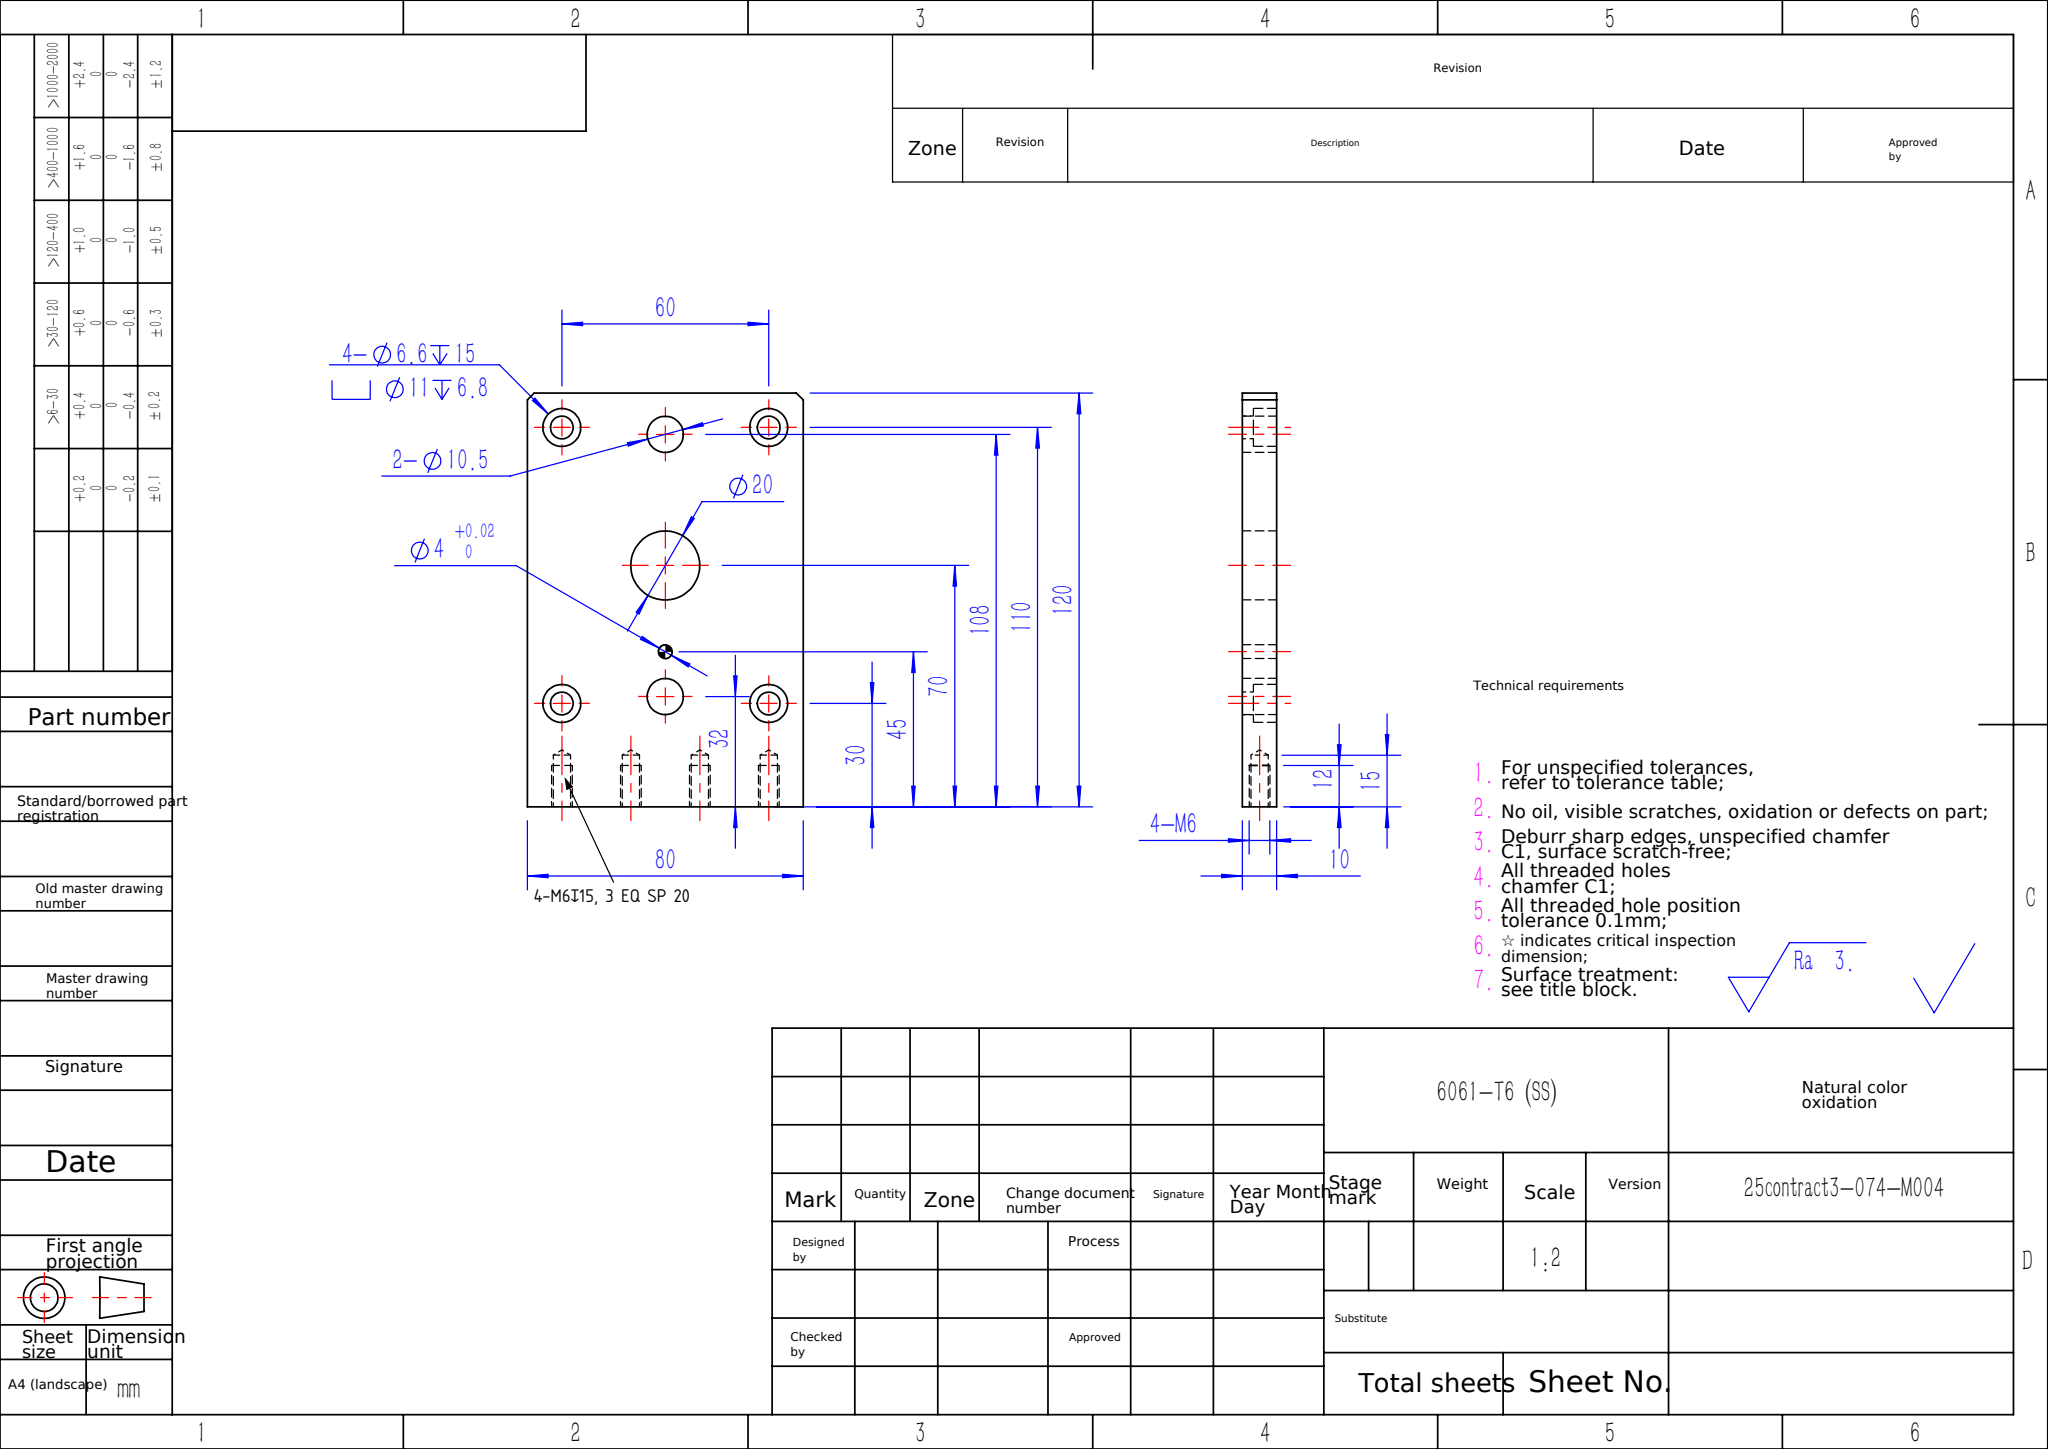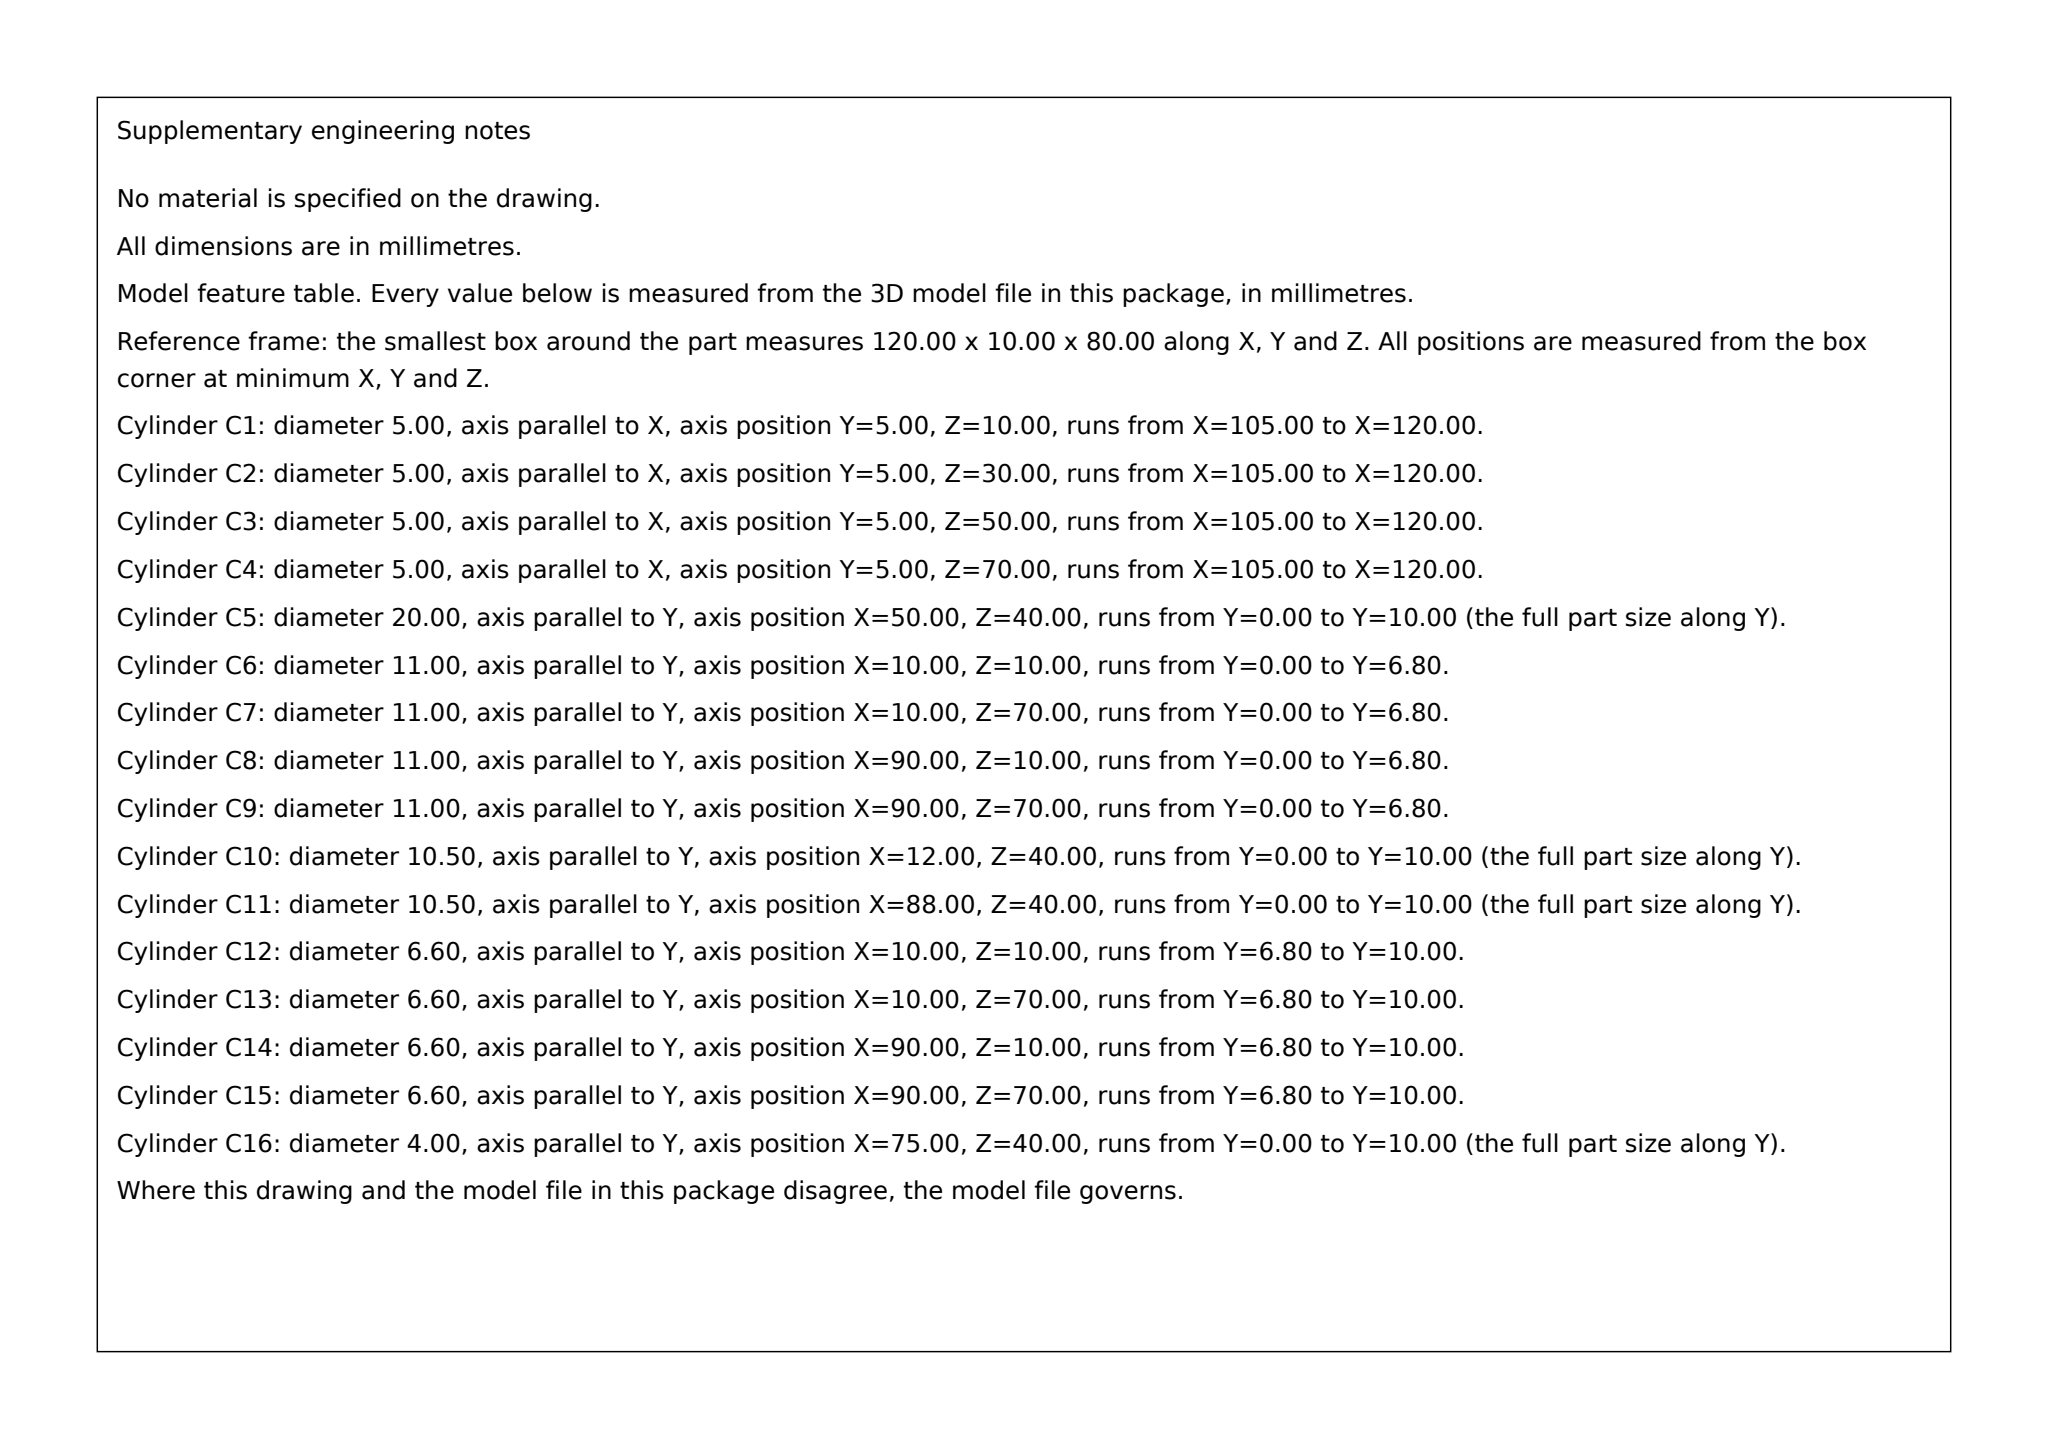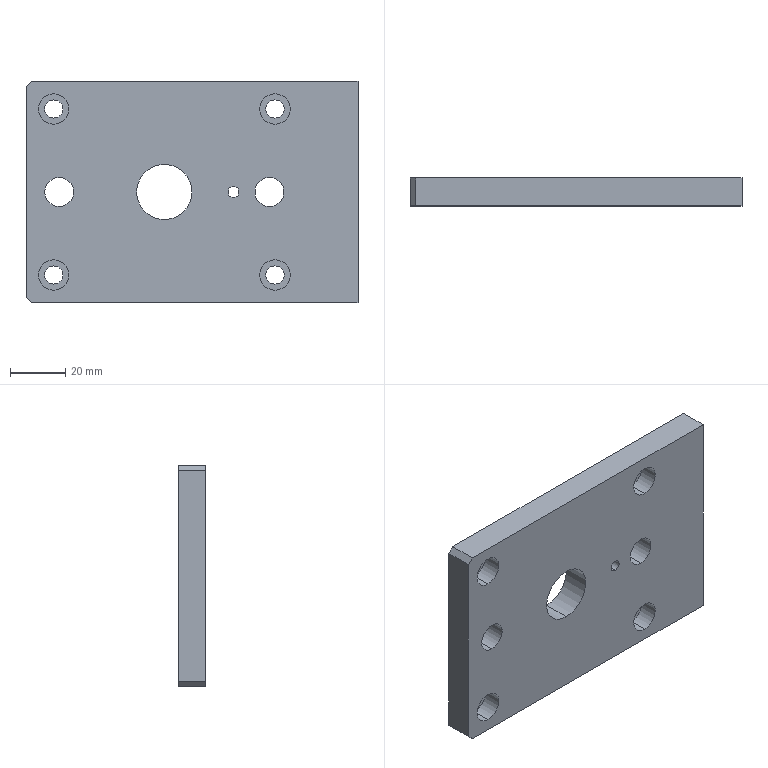Part | SolidWorks | mm | material 6061-T6 (SS) | 1 solid | 52 faces | box 120 x 10 x 80 mm | volume 86721 mm3 | cylinder 32 | plane 12 | cone 8 | commonest cylinder face diameters 11 x8 6.6 x8 5 x8 10.5 x4 4 x2 20 x2
Drawing notes:
4-M6 DP 15: 3 EQ SP 20, END HOLES 10 FROM EACH SIDE EDGE | from the solid: Ø5 x-axis holes, L15, at z=10,30,50,70 (y=5) in 80-wide part
build123d program:
from build123d import *

# Parameters (mm, degrees)
SKETCH1_W                                         = 120
SKETCH1_H                                         = 80
SKETCH1_R                                         = 10
BOSS_EXTRUDE1_DEPTH                               = 10
F_10_5_10_5_DIAMETER_HOLE1_D                      = 10.5
F_10_5_10_5_DIAMETER_HOLE1_DEPTH                  = 15
F_10_5_10_5_DIAMETER_HOLE1_TIP                    = 3.155
SIZE_MM_DOWEL_PIN_HOLE1_D                         = 4
SIZE_MM_DOWEL_PIN_HOLE1_DEPTH                     = 15
SIZE_MM_DOWEL_PIN_HOLE1_TIP                       = 1.202
M6_TAPPED_HOLE1_D                                 = 5
M6_TAPPED_HOLE1_DEPTH                             = 15
M6_TAPPED_HOLE1_TIP                               = 1.502
HOLE_SIZE_ACCORDING_TO_HEXAGON_SOCKET_D           = 6.6
HOLE_SIZE_ACCORDING_TO_HEXAGON_SOCKET_DEPTH       = 15
HOLE_SIZE_ACCORDING_TO_HEXAGON_SOCKET_CBORE_D     = 11
HOLE_SIZE_ACCORDING_TO_HEXAGON_SOCKET_CBORE_DEPTH = 6.8
HOLE_SIZE_ACCORDING_TO_HEXAGON_SOCKET_TIP         = 1.983
CHAMFER2_SIZE                                     = 2


with BuildPart() as part:
    # Sketch1 → Boss-Extrude1 (new body)
    with BuildSketch(Plane(origin=(0, 0, 0), x_dir=(1, 0, 0), z_dir=(0, 1, 0))):
        Rectangle(SKETCH1_W, SKETCH1_H)
        with Locations(Location((-10, 0, 0), (0, 0, 270))):
            Circle(SKETCH1_R, mode=Mode.SUBTRACT)
    extrude(amount=BOSS_EXTRUDE1_DEPTH)

    # 10.5 _10.5_ Diameter Hole1
    with Locations(Plane(origin=(0, 10, 0), x_dir=(1, 0, 0), z_dir=(0, 1, 0))):
        with Locations((-48, 0), (28, 0)):
            Hole(F_10_5_10_5_DIAMETER_HOLE1_D / 2, depth=F_10_5_10_5_DIAMETER_HOLE1_DEPTH)
            with Locations((0, 0, -(F_10_5_10_5_DIAMETER_HOLE1_DEPTH + F_10_5_10_5_DIAMETER_HOLE1_TIP / 2))):  # 118° drill point
                Cone(0, F_10_5_10_5_DIAMETER_HOLE1_D / 2, F_10_5_10_5_DIAMETER_HOLE1_TIP, mode=Mode.SUBTRACT)

    # Size mm Dowel Pin Hole1
    with Locations(Plane(origin=(0, 10, 0), x_dir=(1, 0, 0), z_dir=(0, 1, 0))):
        with Locations((15, 0)):
            Hole(SIZE_MM_DOWEL_PIN_HOLE1_D / 2, depth=SIZE_MM_DOWEL_PIN_HOLE1_DEPTH)
            with Locations((0, 0, -(SIZE_MM_DOWEL_PIN_HOLE1_DEPTH + SIZE_MM_DOWEL_PIN_HOLE1_TIP / 2))):  # 118° drill point
                Cone(0, SIZE_MM_DOWEL_PIN_HOLE1_D / 2, SIZE_MM_DOWEL_PIN_HOLE1_TIP, mode=Mode.SUBTRACT)

    # M6 Tapped Hole1
    with Locations(Plane(origin=(60, 0, 0), x_dir=(0, 0, -1), z_dir=(1, 0, 0))):
        with Locations((30, 5), (10, 5), (-10, 5), (-30, 5)):
            Hole(M6_TAPPED_HOLE1_D / 2, depth=M6_TAPPED_HOLE1_DEPTH)
            with Locations((0, 0, -(M6_TAPPED_HOLE1_DEPTH + M6_TAPPED_HOLE1_TIP / 2))):  # 118° drill point
                Cone(0, M6_TAPPED_HOLE1_D / 2, M6_TAPPED_HOLE1_TIP, mode=Mode.SUBTRACT)

    # Hole Size _ according to_ Hexagon Socket
    with Locations(Plane(origin=(0, 0, 0), x_dir=(-1, 0, 0), z_dir=(0, -1, 0))):
        with Locations((50, 30), (-30, 30), (-30, -30), (50, -30)):
            CounterBoreHole(HOLE_SIZE_ACCORDING_TO_HEXAGON_SOCKET_D / 2, HOLE_SIZE_ACCORDING_TO_HEXAGON_SOCKET_CBORE_D / 2, HOLE_SIZE_ACCORDING_TO_HEXAGON_SOCKET_CBORE_DEPTH, depth=HOLE_SIZE_ACCORDING_TO_HEXAGON_SOCKET_DEPTH)
            with Locations((0, 0, -(HOLE_SIZE_ACCORDING_TO_HEXAGON_SOCKET_DEPTH + HOLE_SIZE_ACCORDING_TO_HEXAGON_SOCKET_TIP / 2))):  # 118° drill point
                Cone(0, HOLE_SIZE_ACCORDING_TO_HEXAGON_SOCKET_D / 2, HOLE_SIZE_ACCORDING_TO_HEXAGON_SOCKET_TIP, mode=Mode.SUBTRACT)

    # Chamfer2
    chamfer2_edges = [part.edges().sort_by_distance(p)[0] for p in [
        (-60, 5, 40),
        (-60, 5, -40),
    ]]
    chamfer(chamfer2_edges, length=CHAMFER2_SIZE)


solid = part.part